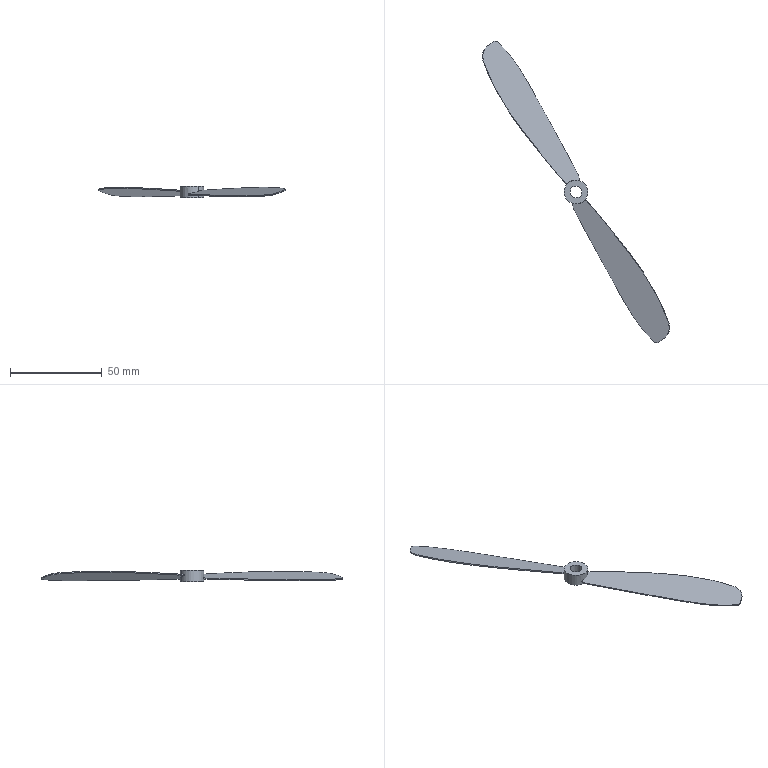Component | SolidWorks | FanBlade-3 | 1 solid | 22 faces | box 102.14 x 164.79 x 6.5 mm | volume 2171 mm3 | cylinder 8 | plane 8 | spline 6 | commonest cylinder face diameters 6.5 x2 13 x2 16 x2 4 x2
STEP:
#1=COLOUR_RGB('',0.7922,0.8196,0.9333);
#2=FILL_AREA_STYLE_COLOUR('',#1);
#3=FILL_AREA_STYLE('',(#2));
#4=SURFACE_STYLE_FILL_AREA(#3);
#5=SURFACE_SIDE_STYLE('',(#4));
#6=SURFACE_STYLE_USAGE(.BOTH.,#5);
#7=PRESENTATION_STYLE_ASSIGNMENT((#6));
#8=CARTESIAN_POINT('',(7.222,3.864,42.691));
#9=VERTEX_POINT('',#8);
#10=CARTESIAN_POINT('',(7.355,3.645,42.691));
#11=VERTEX_POINT('',#10);
#12=CARTESIAN_POINT('',(7.289,3.755,42.691));
#13=DIRECTION('',(-0.,-0.,1.));
#14=DIRECTION('',(0.521,-0.8535,0.));
#15=AXIS2_PLACEMENT_3D('',#12,#13,#14);
#16=CIRCLE('',#15,0.128);
#17=EDGE_CURVE('',#9,#11,#16,.T.);
#18=ORIENTED_EDGE('',*,*,#17,.F.);
#19=CARTESIAN_POINT('',(7.222,3.864,42.947));
#20=VERTEX_POINT('',#19);
#21=CARTESIAN_POINT('',(7.222,3.864,42.348));
#22=DIRECTION('',(-0.,-0.,1.));
#23=VECTOR('',#22,39.37);
#24=LINE('',#21,#23);
#25=EDGE_CURVE('',#9,#20,#24,.T.);
#26=ORIENTED_EDGE('',*,*,#25,.T.);
#27=CARTESIAN_POINT('',(7.355,3.645,42.947));
#28=VERTEX_POINT('',#27);
#29=CARTESIAN_POINT('',(7.289,3.755,42.947));
#30=DIRECTION('',(-0.,-0.,1.));
#31=DIRECTION('',(0.521,-0.8535,0.));
#32=AXIS2_PLACEMENT_3D('',#29,#30,#31);
#33=CIRCLE('',#32,0.128);
#34=EDGE_CURVE('',#20,#28,#33,.T.);
#35=ORIENTED_EDGE('',*,*,#34,.T.);
#36=CARTESIAN_POINT('',(7.355,3.645,42.348));
#37=DIRECTION('',(-0.,-0.,1.));
#38=VECTOR('',#37,39.37);
#39=LINE('',#36,#38);
#40=EDGE_CURVE('',#11,#28,#39,.T.);
#41=ORIENTED_EDGE('',*,*,#40,.F.);
#42=EDGE_LOOP('',(#18,#26,#35,#41));
#43=FACE_OUTER_BOUND('',#42,.T.);
#44=CARTESIAN_POINT('',(7.289,3.755,42.348));
#45=DIRECTION('',(-0.,-0.,1.));
#46=DIRECTION('',(0.521,-0.8535,0.));
#47=AXIS2_PLACEMENT_3D('',#44,#45,#46);
#48=CYLINDRICAL_SURFACE('',#47,0.128);
#49=ADVANCED_FACE('',(#43),#48,.F.);
#50=CARTESIAN_POINT('',(7.422,3.536,42.947));
#51=VERTEX_POINT('',#50);
#52=CARTESIAN_POINT('',(7.155,3.973,42.947));
#53=VERTEX_POINT('',#52);
#54=CARTESIAN_POINT('',(7.289,3.755,42.947));
#55=DIRECTION('',(-0.,-0.,1.));
#56=DIRECTION('',(0.521,-0.8535,0.));
#57=AXIS2_PLACEMENT_3D('',#54,#55,#56);
#58=CIRCLE('',#57,0.2559);
#59=EDGE_CURVE('',#51,#53,#58,.T.);
#60=ORIENTED_EDGE('',*,*,#59,.F.);
#61=CARTESIAN_POINT('',(7.422,3.536,42.831));
#62=VERTEX_POINT('',#61);
#63=CARTESIAN_POINT('',(7.422,3.536,42.947));
#64=DIRECTION('',(0.,0.,-1.));
#65=VECTOR('',#64,39.37);
#66=LINE('',#63,#65);
#67=EDGE_CURVE('',#51,#62,#66,.T.);
#68=ORIENTED_EDGE('',*,*,#67,.T.);
#69=CARTESIAN_POINT('',(7.48,3.585,42.851));
#70=VERTEX_POINT('',#69);
#71=CARTESIAN_POINT('',(7.422,3.536,42.831));
#72=CARTESIAN_POINT('',(7.444,3.55,42.838));
#73=CARTESIAN_POINT('',(7.463,3.566,42.845));
#74=CARTESIAN_POINT('',(7.48,3.585,42.851));
#75=(BOUNDED_CURVE()B_SPLINE_CURVE(3,(#71,#72,#73,#74),.UNSPECIFIED.,.F.,.F.)B_SPLINE_CURVE_WITH_KNOTS((4,4),(1.571,1.87),.UNSPECIFIED.)CURVE()GEOMETRIC_REPRESENTATION_ITEM()RATIONAL_B_SPLINE_CURVE((1.,0.9926,0.9926,1.))REPRESENTATION_ITEM(''));
#76=EDGE_CURVE('',#62,#70,#75,.T.);
#77=ORIENTED_EDGE('',*,*,#76,.T.);
#78=CARTESIAN_POINT('',(7.484,3.59,42.828));
#79=VERTEX_POINT('',#78);
#80=CARTESIAN_POINT('',(7.484,3.59,42.828));
#81=CARTESIAN_POINT('',(7.483,3.588,42.836));
#82=CARTESIAN_POINT('',(7.482,3.587,42.844));
#83=CARTESIAN_POINT('',(7.48,3.585,42.851));
#84=B_SPLINE_CURVE_WITH_KNOTS('',3,(#80,#81,#82,#83),.UNSPECIFIED.,.F.,.F.,(4,4),(0.,0.0006019),.UNSPECIFIED.);
#85=EDGE_CURVE('',#79,#70,#84,.T.);
#86=ORIENTED_EDGE('',*,*,#85,.F.);
#87=CARTESIAN_POINT('',(7.422,3.536,42.807));
#88=VERTEX_POINT('',#87);
#89=CARTESIAN_POINT('',(7.422,3.536,42.807));
#90=CARTESIAN_POINT('',(7.445,3.551,42.814));
#91=CARTESIAN_POINT('',(7.466,3.568,42.821));
#92=CARTESIAN_POINT('',(7.484,3.59,42.828));
#93=(BOUNDED_CURVE()B_SPLINE_CURVE(3,(#89,#90,#91,#92),.UNSPECIFIED.,.F.,.T.)B_SPLINE_CURVE_WITH_KNOTS((4,4),(1.571,1.892),.UNSPECIFIED.)CURVE()GEOMETRIC_REPRESENTATION_ITEM()RATIONAL_B_SPLINE_CURVE((1.,0.9914,0.9914,1.))REPRESENTATION_ITEM(''));
#94=EDGE_CURVE('',#88,#79,#93,.T.);
#95=ORIENTED_EDGE('',*,*,#94,.F.);
#96=CARTESIAN_POINT('',(7.422,3.536,42.691));
#97=VERTEX_POINT('',#96);
#98=CARTESIAN_POINT('',(7.422,3.536,42.947));
#99=DIRECTION('',(0.,0.,-1.));
#100=VECTOR('',#99,39.37);
#101=LINE('',#98,#100);
#102=EDGE_CURVE('',#88,#97,#101,.T.);
#103=ORIENTED_EDGE('',*,*,#102,.T.);
#104=CARTESIAN_POINT('',(7.155,3.973,42.691));
#105=VERTEX_POINT('',#104);
#106=CARTESIAN_POINT('',(7.289,3.755,42.691));
#107=DIRECTION('',(-0.,-0.,1.));
#108=DIRECTION('',(0.521,-0.8535,0.));
#109=AXIS2_PLACEMENT_3D('',#106,#107,#108);
#110=CIRCLE('',#109,0.2559);
#111=EDGE_CURVE('',#97,#105,#110,.T.);
#112=ORIENTED_EDGE('',*,*,#111,.T.);
#113=CARTESIAN_POINT('',(7.155,3.973,42.807));
#114=VERTEX_POINT('',#113);
#115=CARTESIAN_POINT('',(7.155,3.973,42.947));
#116=DIRECTION('',(0.,0.,-1.));
#117=VECTOR('',#116,39.37);
#118=LINE('',#115,#117);
#119=EDGE_CURVE('',#114,#105,#118,.T.);
#120=ORIENTED_EDGE('',*,*,#119,.F.);
#121=CARTESIAN_POINT('',(7.363,4.,42.756));
#122=VERTEX_POINT('',#121);
#123=CARTESIAN_POINT('',(7.363,4.,42.756));
#124=CARTESIAN_POINT('',(7.292,4.021,42.769));
#125=CARTESIAN_POINT('',(7.218,4.012,42.787));
#126=CARTESIAN_POINT('',(7.155,3.973,42.807));
#127=(BOUNDED_CURVE()B_SPLINE_CURVE(3,(#123,#124,#125,#126),.UNSPECIFIED.,.F.,.T.)B_SPLINE_CURVE_WITH_KNOTS((4,4),(0.7294,1.571),.UNSPECIFIED.)CURVE()GEOMETRIC_REPRESENTATION_ITEM()RATIONAL_B_SPLINE_CURVE((1.,0.9419,0.9419,1.))REPRESENTATION_ITEM(''));
#128=EDGE_CURVE('',#122,#114,#127,.T.);
#129=ORIENTED_EDGE('',*,*,#128,.F.);
#130=CARTESIAN_POINT('',(7.368,3.998,42.779));
#131=VERTEX_POINT('',#130);
#132=CARTESIAN_POINT('',(7.368,3.998,42.779));
#133=CARTESIAN_POINT('',(7.366,3.998,42.771));
#134=CARTESIAN_POINT('',(7.364,3.999,42.763));
#135=CARTESIAN_POINT('',(7.363,4.,42.756));
#136=(BOUNDED_CURVE()B_SPLINE_CURVE(3,(#132,#133,#134,#135),.UNSPECIFIED.,.F.,.T.)B_SPLINE_CURVE_WITH_KNOTS((4,4),(4.388,4.41),.UNSPECIFIED.)CURVE()GEOMETRIC_REPRESENTATION_ITEM()RATIONAL_B_SPLINE_CURVE((1.,1.,1.,1.))REPRESENTATION_ITEM(''));
#137=EDGE_CURVE('',#131,#122,#136,.T.);
#138=ORIENTED_EDGE('',*,*,#137,.F.);
#139=CARTESIAN_POINT('',(7.155,3.973,42.831));
#140=VERTEX_POINT('',#139);
#141=CARTESIAN_POINT('',(7.368,3.998,42.779));
#142=CARTESIAN_POINT('',(7.296,4.021,42.792));
#143=CARTESIAN_POINT('',(7.22,4.013,42.811));
#144=CARTESIAN_POINT('',(7.155,3.973,42.831));
#145=(BOUNDED_CURVE()B_SPLINE_CURVE(3,(#141,#142,#143,#144),.UNSPECIFIED.,.F.,.T.)B_SPLINE_CURVE_WITH_KNOTS((4,4),(0.7073,1.571),.UNSPECIFIED.)CURVE()GEOMETRIC_REPRESENTATION_ITEM()RATIONAL_B_SPLINE_CURVE((1.,0.9388,0.9388,1.))REPRESENTATION_ITEM(''));
#146=EDGE_CURVE('',#131,#140,#145,.T.);
#147=ORIENTED_EDGE('',*,*,#146,.T.);
#148=CARTESIAN_POINT('',(7.155,3.973,42.947));
#149=DIRECTION('',(0.,0.,-1.));
#150=VECTOR('',#149,39.37);
#151=LINE('',#148,#150);
#152=EDGE_CURVE('',#53,#140,#151,.T.);
#153=ORIENTED_EDGE('',*,*,#152,.F.);
#154=EDGE_LOOP('',(#60,#68,#77,#86,#95,#103,#112,#120,#129,#138,#147,#153));
#155=FACE_OUTER_BOUND('',#154,.T.);
#156=CARTESIAN_POINT('',(7.289,3.755,42.947));
#157=DIRECTION('',(0.,0.,-1.));
#158=DIRECTION('',(-0.521,0.8535,0.));
#159=AXIS2_PLACEMENT_3D('',#156,#157,#158);
#160=CYLINDRICAL_SURFACE('',#159,0.2559);
#161=ADVANCED_FACE('',(#155),#160,.T.);
#162=ORIENTED_EDGE('',*,*,#67,.F.);
#163=CARTESIAN_POINT('',(7.289,3.755,42.947));
#164=DIRECTION('',(-0.,-0.,1.));
#165=DIRECTION('',(0.521,-0.8535,0.));
#166=AXIS2_PLACEMENT_3D('',#163,#164,#165);
#167=CIRCLE('',#166,0.2559);
#168=EDGE_CURVE('',#53,#51,#167,.T.);
#169=ORIENTED_EDGE('',*,*,#168,.F.);
#170=ORIENTED_EDGE('',*,*,#152,.T.);
#171=CARTESIAN_POINT('',(7.097,3.924,42.851));
#172=VERTEX_POINT('',#171);
#173=CARTESIAN_POINT('',(7.155,3.973,42.831));
#174=CARTESIAN_POINT('',(7.133,3.96,42.838));
#175=CARTESIAN_POINT('',(7.114,3.943,42.845));
#176=CARTESIAN_POINT('',(7.097,3.924,42.851));
#177=(BOUNDED_CURVE()B_SPLINE_CURVE(3,(#173,#174,#175,#176),.UNSPECIFIED.,.F.,.F.)B_SPLINE_CURVE_WITH_KNOTS((4,4),(1.571,1.87),.UNSPECIFIED.)CURVE()GEOMETRIC_REPRESENTATION_ITEM()RATIONAL_B_SPLINE_CURVE((1.,0.9926,0.9926,1.))REPRESENTATION_ITEM(''));
#178=EDGE_CURVE('',#140,#172,#177,.T.);
#179=ORIENTED_EDGE('',*,*,#178,.T.);
#180=CARTESIAN_POINT('',(7.093,3.92,42.828));
#181=VERTEX_POINT('',#180);
#182=CARTESIAN_POINT('',(7.093,3.92,42.828));
#183=CARTESIAN_POINT('',(7.094,3.921,42.836));
#184=CARTESIAN_POINT('',(7.095,3.923,42.844));
#185=CARTESIAN_POINT('',(7.097,3.924,42.851));
#186=B_SPLINE_CURVE_WITH_KNOTS('',3,(#182,#183,#184,#185),.UNSPECIFIED.,.F.,.F.,(4,4),(0.,0.0006019),.UNSPECIFIED.);
#187=EDGE_CURVE('',#181,#172,#186,.T.);
#188=ORIENTED_EDGE('',*,*,#187,.F.);
#189=CARTESIAN_POINT('',(7.155,3.973,42.807));
#190=CARTESIAN_POINT('',(7.132,3.959,42.814));
#191=CARTESIAN_POINT('',(7.111,3.941,42.821));
#192=CARTESIAN_POINT('',(7.093,3.92,42.828));
#193=(BOUNDED_CURVE()B_SPLINE_CURVE(3,(#189,#190,#191,#192),.UNSPECIFIED.,.F.,.T.)B_SPLINE_CURVE_WITH_KNOTS((4,4),(1.571,1.892),.UNSPECIFIED.)CURVE()GEOMETRIC_REPRESENTATION_ITEM()RATIONAL_B_SPLINE_CURVE((1.,0.9914,0.9914,1.))REPRESENTATION_ITEM(''));
#194=EDGE_CURVE('',#114,#181,#193,.T.);
#195=ORIENTED_EDGE('',*,*,#194,.F.);
#196=ORIENTED_EDGE('',*,*,#119,.T.);
#197=CARTESIAN_POINT('',(7.289,3.755,42.691));
#198=DIRECTION('',(-0.,-0.,1.));
#199=DIRECTION('',(0.521,-0.8535,0.));
#200=AXIS2_PLACEMENT_3D('',#197,#198,#199);
#201=CIRCLE('',#200,0.2559);
#202=EDGE_CURVE('',#105,#97,#201,.T.);
#203=ORIENTED_EDGE('',*,*,#202,.T.);
#204=ORIENTED_EDGE('',*,*,#102,.F.);
#205=CARTESIAN_POINT('',(7.215,3.51,42.756));
#206=VERTEX_POINT('',#205);
#207=CARTESIAN_POINT('',(7.215,3.51,42.756));
#208=CARTESIAN_POINT('',(7.285,3.488,42.769));
#209=CARTESIAN_POINT('',(7.359,3.498,42.787));
#210=CARTESIAN_POINT('',(7.422,3.536,42.807));
#211=(BOUNDED_CURVE()B_SPLINE_CURVE(3,(#207,#208,#209,#210),.UNSPECIFIED.,.F.,.T.)B_SPLINE_CURVE_WITH_KNOTS((4,4),(0.7294,1.571),.UNSPECIFIED.)CURVE()GEOMETRIC_REPRESENTATION_ITEM()RATIONAL_B_SPLINE_CURVE((1.,0.9419,0.9419,1.))REPRESENTATION_ITEM(''));
#212=EDGE_CURVE('',#206,#88,#211,.T.);
#213=ORIENTED_EDGE('',*,*,#212,.F.);
#214=CARTESIAN_POINT('',(7.209,3.511,42.779));
#215=VERTEX_POINT('',#214);
#216=CARTESIAN_POINT('',(7.209,3.511,42.779));
#217=CARTESIAN_POINT('',(7.211,3.511,42.771));
#218=CARTESIAN_POINT('',(7.213,3.51,42.763));
#219=CARTESIAN_POINT('',(7.215,3.51,42.756));
#220=(BOUNDED_CURVE()B_SPLINE_CURVE(3,(#216,#217,#218,#219),.UNSPECIFIED.,.F.,.T.)B_SPLINE_CURVE_WITH_KNOTS((4,4),(4.388,4.41),.UNSPECIFIED.)CURVE()GEOMETRIC_REPRESENTATION_ITEM()RATIONAL_B_SPLINE_CURVE((1.,1.,1.,1.))REPRESENTATION_ITEM(''));
#221=EDGE_CURVE('',#215,#206,#220,.T.);
#222=ORIENTED_EDGE('',*,*,#221,.F.);
#223=CARTESIAN_POINT('',(7.209,3.511,42.779));
#224=CARTESIAN_POINT('',(7.281,3.488,42.792));
#225=CARTESIAN_POINT('',(7.357,3.497,42.811));
#226=CARTESIAN_POINT('',(7.422,3.536,42.831));
#227=(BOUNDED_CURVE()B_SPLINE_CURVE(3,(#223,#224,#225,#226),.UNSPECIFIED.,.F.,.T.)B_SPLINE_CURVE_WITH_KNOTS((4,4),(0.7073,1.571),.UNSPECIFIED.)CURVE()GEOMETRIC_REPRESENTATION_ITEM()RATIONAL_B_SPLINE_CURVE((1.,0.9388,0.9388,1.))REPRESENTATION_ITEM(''));
#228=EDGE_CURVE('',#215,#62,#227,.T.);
#229=ORIENTED_EDGE('',*,*,#228,.T.);
#230=EDGE_LOOP('',(#162,#169,#170,#179,#188,#195,#196,#203,#204,#213,#222,#229));
#231=FACE_OUTER_BOUND('',#230,.T.);
#232=CARTESIAN_POINT('',(7.289,3.755,42.947));
#233=DIRECTION('',(0.,0.,-1.));
#234=DIRECTION('',(-0.521,0.8535,0.));
#235=AXIS2_PLACEMENT_3D('',#232,#233,#234);
#236=CYLINDRICAL_SURFACE('',#235,0.2559);
#237=ADVANCED_FACE('',(#231),#236,.T.);
#238=CARTESIAN_POINT('',(7.289,3.755,42.947));
#239=DIRECTION('',(-0.,-0.,1.));
#240=DIRECTION('',(0.521,-0.8535,0.));
#241=AXIS2_PLACEMENT_3D('',#238,#239,#240);
#242=CIRCLE('',#241,0.128);
#243=EDGE_CURVE('',#28,#20,#242,.T.);
#244=ORIENTED_EDGE('',*,*,#243,.F.);
#245=ORIENTED_EDGE('',*,*,#34,.F.);
#246=EDGE_LOOP('',(#244,#245));
#247=FACE_BOUND('',#246,.T.);
#248=ORIENTED_EDGE('',*,*,#168,.T.);
#249=ORIENTED_EDGE('',*,*,#59,.T.);
#250=EDGE_LOOP('',(#248,#249));
#251=FACE_OUTER_BOUND('',#250,.T.);
#252=CARTESIAN_POINT('',(7.289,3.755,42.947));
#253=DIRECTION('',(-0.,-0.,1.));
#254=DIRECTION('',(0.521,-0.8535,0.));
#255=AXIS2_PLACEMENT_3D('',#252,#253,#254);
#256=PLANE('',#255);
#257=ADVANCED_FACE('',(#247,#251),#256,.T.);
#258=CARTESIAN_POINT('',(7.289,3.755,42.691));
#259=DIRECTION('',(-0.,-0.,1.));
#260=DIRECTION('',(0.521,-0.8535,0.));
#261=AXIS2_PLACEMENT_3D('',#258,#259,#260);
#262=CIRCLE('',#261,0.128);
#263=EDGE_CURVE('',#11,#9,#262,.T.);
#264=ORIENTED_EDGE('',*,*,#263,.T.);
#265=ORIENTED_EDGE('',*,*,#17,.T.);
#266=EDGE_LOOP('',(#264,#265));
#267=FACE_BOUND('',#266,.T.);
#268=ORIENTED_EDGE('',*,*,#202,.F.);
#269=ORIENTED_EDGE('',*,*,#111,.F.);
#270=EDGE_LOOP('',(#268,#269));
#271=FACE_OUTER_BOUND('',#270,.T.);
#272=CARTESIAN_POINT('',(7.289,3.755,42.691));
#273=DIRECTION('',(-0.,-0.,1.));
#274=DIRECTION('',(0.521,-0.8535,0.));
#275=AXIS2_PLACEMENT_3D('',#272,#273,#274);
#276=PLANE('',#275);
#277=ADVANCED_FACE('',(#267,#271),#276,.F.);
#278=CARTESIAN_POINT('',(9.29,0.9176,42.868));
#279=VERTEX_POINT('',#278);
#280=CARTESIAN_POINT('',(7.484,3.59,42.828));
#281=CARTESIAN_POINT('',(7.594,3.497,42.84));
#282=CARTESIAN_POINT('',(8.277,2.647,42.878));
#283=CARTESIAN_POINT('',(8.978,1.852,42.927));
#284=CARTESIAN_POINT('',(9.29,0.9176,42.868));
#285=B_SPLINE_CURVE_WITH_KNOTS('',3,(#280,#281,#282,#283,#284),.UNSPECIFIED.,.F.,.F.,(4,1,4),(0.05263,0.18,1.),.UNSPECIFIED.);
#286=EDGE_CURVE('',#79,#279,#285,.T.);
#287=ORIENTED_EDGE('',*,*,#286,.F.);
#288=ORIENTED_EDGE('',*,*,#85,.T.);
#289=CARTESIAN_POINT('',(9.285,0.9144,42.891));
#290=VERTEX_POINT('',#289);
#291=CARTESIAN_POINT('',(7.48,3.585,42.851));
#292=CARTESIAN_POINT('',(7.589,3.492,42.863));
#293=CARTESIAN_POINT('',(8.272,2.643,42.901));
#294=CARTESIAN_POINT('',(8.973,1.848,42.95));
#295=CARTESIAN_POINT('',(9.285,0.9144,42.891));
#296=B_SPLINE_CURVE_WITH_KNOTS('',3,(#291,#292,#293,#294,#295),.UNSPECIFIED.,.F.,.F.,(4,1,4),(0.05318,0.18,1.),.UNSPECIFIED.);
#297=EDGE_CURVE('',#70,#290,#296,.T.);
#298=ORIENTED_EDGE('',*,*,#297,.T.);
#299=CARTESIAN_POINT('',(9.29,0.9176,42.868));
#300=DIRECTION('',(-0.2209,-0.1349,0.9659));
#301=VECTOR('',#300,39.37);
#302=LINE('',#299,#301);
#303=EDGE_CURVE('',#279,#290,#302,.T.);
#304=ORIENTED_EDGE('',*,*,#303,.F.);
#305=EDGE_LOOP('',(#287,#288,#298,#304));
#306=FACE_OUTER_BOUND('',#305,.T.);
#307=CARTESIAN_POINT('',(7.469,3.602,42.827));
#308=CARTESIAN_POINT('',(7.464,3.599,42.849));
#309=CARTESIAN_POINT('',(7.586,3.507,42.84));
#310=CARTESIAN_POINT('',(7.58,3.504,42.863));
#311=CARTESIAN_POINT('',(8.272,2.651,42.878));
#312=CARTESIAN_POINT('',(8.267,2.648,42.9));
#313=CARTESIAN_POINT('',(8.978,1.852,42.927));
#314=CARTESIAN_POINT('',(8.973,1.848,42.95));
#315=CARTESIAN_POINT('',(9.29,0.9176,42.868));
#316=CARTESIAN_POINT('',(9.285,0.9144,42.891));
#317=B_SPLINE_SURFACE_WITH_KNOTS('',3,1,((#307,#308),(#309,#310),(#311,#312),(#313,#314),(#315,#316)),.UNSPECIFIED.,.F.,.F.,.F.,(4,1,4),(2,2),(0.04695,0.18,1.),(0.,1.),.UNSPECIFIED.);
#318=ADVANCED_FACE('',(#306),#317,.F.);
#319=CARTESIAN_POINT('',(8.961,0.5322,42.764));
#320=VERTEX_POINT('',#319);
#321=CARTESIAN_POINT('',(7.257,3.349,42.767));
#322=VERTEX_POINT('',#321);
#323=CARTESIAN_POINT('',(8.961,0.5322,42.764));
#324=CARTESIAN_POINT('',(8.664,0.8114,42.735));
#325=CARTESIAN_POINT('',(8.095,1.779,42.74));
#326=CARTESIAN_POINT('',(7.587,2.738,42.757));
#327=CARTESIAN_POINT('',(7.257,3.349,42.767));
#328=B_SPLINE_CURVE_WITH_KNOTS('',3,(#323,#324,#325,#326,#327),.UNSPECIFIED.,.F.,.F.,(4,1,4),(0.,0.3608,0.9726),.UNSPECIFIED.);
#329=EDGE_CURVE('',#320,#322,#328,.T.);
#330=ORIENTED_EDGE('',*,*,#329,.T.);
#331=CARTESIAN_POINT('',(7.262,3.353,42.744));
#332=VERTEX_POINT('',#331);
#333=CARTESIAN_POINT('',(7.257,3.349,42.767));
#334=CARTESIAN_POINT('',(7.258,3.35,42.76));
#335=CARTESIAN_POINT('',(7.26,3.351,42.752));
#336=CARTESIAN_POINT('',(7.262,3.353,42.744));
#337=B_SPLINE_CURVE_WITH_KNOTS('',3,(#333,#334,#335,#336),.UNSPECIFIED.,.F.,.F.,(4,4),(0.,0.0006001),.UNSPECIFIED.);
#338=EDGE_CURVE('',#322,#332,#337,.T.);
#339=ORIENTED_EDGE('',*,*,#338,.T.);
#340=CARTESIAN_POINT('',(8.967,0.5354,42.741));
#341=VERTEX_POINT('',#340);
#342=CARTESIAN_POINT('',(8.967,0.5354,42.741));
#343=CARTESIAN_POINT('',(8.669,0.8146,42.712));
#344=CARTESIAN_POINT('',(8.101,1.782,42.717));
#345=CARTESIAN_POINT('',(7.592,2.742,42.735));
#346=CARTESIAN_POINT('',(7.262,3.353,42.744));
#347=B_SPLINE_CURVE_WITH_KNOTS('',3,(#342,#343,#344,#345,#346),.UNSPECIFIED.,.F.,.F.,(4,1,4),(0.,0.3608,0.9727),.UNSPECIFIED.);
#348=EDGE_CURVE('',#341,#332,#347,.T.);
#349=ORIENTED_EDGE('',*,*,#348,.F.);
#350=CARTESIAN_POINT('',(8.967,0.5354,42.741));
#351=DIRECTION('',(-0.2209,-0.1349,0.9659));
#352=VECTOR('',#351,39.37);
#353=LINE('',#350,#352);
#354=EDGE_CURVE('',#341,#320,#353,.T.);
#355=ORIENTED_EDGE('',*,*,#354,.T.);
#356=EDGE_LOOP('',(#330,#339,#349,#355));
#357=FACE_OUTER_BOUND('',#356,.T.);
#358=CARTESIAN_POINT('',(8.967,0.5354,42.741));
#359=CARTESIAN_POINT('',(8.961,0.5322,42.764));
#360=CARTESIAN_POINT('',(8.669,0.8146,42.712));
#361=CARTESIAN_POINT('',(8.664,0.8114,42.735));
#362=CARTESIAN_POINT('',(8.097,1.788,42.717));
#363=CARTESIAN_POINT('',(8.092,1.785,42.74));
#364=CARTESIAN_POINT('',(7.586,2.753,42.735));
#365=CARTESIAN_POINT('',(7.581,2.75,42.758));
#366=CARTESIAN_POINT('',(7.252,3.37,42.745));
#367=CARTESIAN_POINT('',(7.247,3.367,42.768));
#368=B_SPLINE_SURFACE_WITH_KNOTS('',3,1,((#358,#359),(#360,#361),(#362,#363),(#364,#365),(#366,#367)),.UNSPECIFIED.,.F.,.F.,.F.,(4,1,4),(2,2),(0.,0.3608,0.9785),(0.,1.),.UNSPECIFIED.);
#369=ADVANCED_FACE('',(#357),#368,.F.);
#370=CARTESIAN_POINT('',(9.151,0.581,42.814));
#371=VERTEX_POINT('',#370);
#372=CARTESIAN_POINT('',(8.987,0.8499,42.814));
#373=DIRECTION('',(0.2209,0.1349,-0.9659));
#374=DIRECTION('',(0.8245,0.5033,0.2588));
#375=AXIS2_PLACEMENT_3D('',#372,#373,#374);
#376=CIRCLE('',#375,0.315);
#377=EDGE_CURVE('',#290,#371,#376,.T.);
#378=ORIENTED_EDGE('',*,*,#377,.T.);
#379=CARTESIAN_POINT('',(9.156,0.5842,42.791));
#380=VERTEX_POINT('',#379);
#381=CARTESIAN_POINT('',(9.156,0.5842,42.791));
#382=DIRECTION('',(-0.2209,-0.1349,0.9659));
#383=VECTOR('',#382,39.37);
#384=LINE('',#381,#383);
#385=EDGE_CURVE('',#380,#371,#384,.T.);
#386=ORIENTED_EDGE('',*,*,#385,.F.);
#387=CARTESIAN_POINT('',(8.992,0.853,42.791));
#388=DIRECTION('',(0.2209,0.1349,-0.9659));
#389=DIRECTION('',(0.8245,0.5033,0.2588));
#390=AXIS2_PLACEMENT_3D('',#387,#388,#389);
#391=CIRCLE('',#390,0.315);
#392=EDGE_CURVE('',#279,#380,#391,.T.);
#393=ORIENTED_EDGE('',*,*,#392,.F.);
#394=ORIENTED_EDGE('',*,*,#303,.T.);
#395=EDGE_LOOP('',(#378,#386,#393,#394));
#396=FACE_OUTER_BOUND('',#395,.T.);
#397=CARTESIAN_POINT('',(8.992,0.853,42.791));
#398=DIRECTION('',(-0.2209,-0.1349,0.9659));
#399=DIRECTION('',(-0.8245,-0.5033,-0.2588));
#400=AXIS2_PLACEMENT_3D('',#397,#398,#399);
#401=CYLINDRICAL_SURFACE('',#400,0.315);
#402=ADVANCED_FACE('',(#396),#401,.T.);
#403=CARTESIAN_POINT('',(9.054,0.5216,42.783));
#404=VERTEX_POINT('',#403);
#405=CARTESIAN_POINT('',(9.151,0.581,42.814));
#406=DIRECTION('',(-0.8245,-0.5033,-0.2588));
#407=VECTOR('',#406,39.37);
#408=LINE('',#405,#407);
#409=EDGE_CURVE('',#371,#404,#408,.T.);
#410=ORIENTED_EDGE('',*,*,#409,.T.);
#411=CARTESIAN_POINT('',(9.059,0.5248,42.761));
#412=VERTEX_POINT('',#411);
#413=CARTESIAN_POINT('',(9.059,0.5248,42.761));
#414=DIRECTION('',(-0.2209,-0.1349,0.9659));
#415=VECTOR('',#414,39.37);
#416=LINE('',#413,#415);
#417=EDGE_CURVE('',#412,#404,#416,.T.);
#418=ORIENTED_EDGE('',*,*,#417,.F.);
#419=CARTESIAN_POINT('',(9.156,0.5842,42.791));
#420=DIRECTION('',(-0.8245,-0.5033,-0.2588));
#421=VECTOR('',#420,39.37);
#422=LINE('',#419,#421);
#423=EDGE_CURVE('',#380,#412,#422,.T.);
#424=ORIENTED_EDGE('',*,*,#423,.F.);
#425=ORIENTED_EDGE('',*,*,#385,.T.);
#426=EDGE_LOOP('',(#410,#418,#424,#425));
#427=FACE_OUTER_BOUND('',#426,.T.);
#428=CARTESIAN_POINT('',(9.156,0.5842,42.791));
#429=DIRECTION('',(-0.521,0.8535,-0.));
#430=DIRECTION('',(-0.8535,-0.521,-0.));
#431=AXIS2_PLACEMENT_3D('',#428,#429,#430);
#432=PLANE('',#431);
#433=ADVANCED_FACE('',(#427),#432,.F.);
#434=CARTESIAN_POINT('',(9.012,0.5888,42.783));
#435=DIRECTION('',(0.2209,0.1349,-0.9659));
#436=DIRECTION('',(0.8245,0.5033,0.2588));
#437=AXIS2_PLACEMENT_3D('',#434,#435,#436);
#438=CIRCLE('',#437,0.07874);
#439=EDGE_CURVE('',#404,#320,#438,.T.);
#440=ORIENTED_EDGE('',*,*,#439,.T.);
#441=ORIENTED_EDGE('',*,*,#354,.F.);
#442=CARTESIAN_POINT('',(9.018,0.592,42.761));
#443=DIRECTION('',(0.2209,0.1349,-0.9659));
#444=DIRECTION('',(0.8245,0.5033,0.2588));
#445=AXIS2_PLACEMENT_3D('',#442,#443,#444);
#446=CIRCLE('',#445,0.07874);
#447=EDGE_CURVE('',#412,#341,#446,.T.);
#448=ORIENTED_EDGE('',*,*,#447,.F.);
#449=ORIENTED_EDGE('',*,*,#417,.T.);
#450=EDGE_LOOP('',(#440,#441,#448,#449));
#451=FACE_OUTER_BOUND('',#450,.T.);
#452=CARTESIAN_POINT('',(9.018,0.592,42.761));
#453=DIRECTION('',(-0.2209,-0.1349,0.9659));
#454=DIRECTION('',(-0.8245,-0.5033,-0.2588));
#455=AXIS2_PLACEMENT_3D('',#452,#453,#454);
#456=CYLINDRICAL_SURFACE('',#455,0.07874);
#457=ADVANCED_FACE('',(#451),#456,.T.);
#458=ORIENTED_EDGE('',*,*,#348,.T.);
#459=CARTESIAN_POINT('',(7.262,3.353,42.744));
#460=CARTESIAN_POINT('',(7.249,3.377,42.745));
#461=CARTESIAN_POINT('',(7.238,3.402,42.746));
#462=CARTESIAN_POINT('',(7.226,3.442,42.749));
#463=CARTESIAN_POINT('',(7.223,3.455,42.75));
#464=CARTESIAN_POINT('',(7.218,3.482,42.752));
#465=CARTESIAN_POINT('',(7.216,3.496,42.754));
#466=CARTESIAN_POINT('',(7.215,3.51,42.756));
#467=B_SPLINE_CURVE_WITH_KNOTS('',3,(#459,#460,#461,#462,#463,#464,#465,#466),.UNSPECIFIED.,.F.,.F.,(4,2,2,4),(0.,0.002088,0.003132,0.004176),.UNSPECIFIED.);
#468=EDGE_CURVE('',#332,#206,#467,.T.);
#469=ORIENTED_EDGE('',*,*,#468,.T.);
#470=ORIENTED_EDGE('',*,*,#212,.T.);
#471=ORIENTED_EDGE('',*,*,#94,.T.);
#472=ORIENTED_EDGE('',*,*,#286,.T.);
#473=ORIENTED_EDGE('',*,*,#392,.T.);
#474=ORIENTED_EDGE('',*,*,#423,.T.);
#475=ORIENTED_EDGE('',*,*,#447,.T.);
#476=EDGE_LOOP('',(#458,#469,#470,#471,#472,#473,#474,#475));
#477=FACE_OUTER_BOUND('',#476,.T.);
#478=CARTESIAN_POINT('',(8.024,1.945,42.722));
#479=DIRECTION('',(-0.2209,-0.1349,0.9659));
#480=DIRECTION('',(-0.8245,-0.5033,-0.2588));
#481=AXIS2_PLACEMENT_3D('',#478,#479,#480);
#482=PLANE('',#481);
#483=ADVANCED_FACE('',(#477),#482,.F.);
#484=ORIENTED_EDGE('',*,*,#228,.F.);
#485=CARTESIAN_POINT('',(7.209,3.511,42.779));
#486=CARTESIAN_POINT('',(7.211,3.483,42.776));
#487=CARTESIAN_POINT('',(7.216,3.455,42.773));
#488=CARTESIAN_POINT('',(7.232,3.401,42.769));
#489=CARTESIAN_POINT('',(7.243,3.374,42.768));
#490=CARTESIAN_POINT('',(7.257,3.349,42.767));
#491=B_SPLINE_CURVE_WITH_KNOTS('',3,(#485,#486,#487,#488,#489,#490),.UNSPECIFIED.,.F.,.F.,(4,2,4),(0.,0.002155,0.00431),.UNSPECIFIED.);
#492=EDGE_CURVE('',#215,#322,#491,.T.);
#493=ORIENTED_EDGE('',*,*,#492,.T.);
#494=ORIENTED_EDGE('',*,*,#329,.F.);
#495=ORIENTED_EDGE('',*,*,#439,.F.);
#496=ORIENTED_EDGE('',*,*,#409,.F.);
#497=ORIENTED_EDGE('',*,*,#377,.F.);
#498=ORIENTED_EDGE('',*,*,#297,.F.);
#499=ORIENTED_EDGE('',*,*,#76,.F.);
#500=EDGE_LOOP('',(#484,#493,#494,#495,#496,#497,#498,#499));
#501=FACE_OUTER_BOUND('',#500,.T.);
#502=CARTESIAN_POINT('',(8.019,1.942,42.745));
#503=DIRECTION('',(-0.2209,-0.1349,0.9659));
#504=DIRECTION('',(-0.8245,-0.5033,-0.2588));
#505=AXIS2_PLACEMENT_3D('',#502,#503,#504);
#506=PLANE('',#505);
#507=ADVANCED_FACE('',(#501),#506,.T.);
#508=CARTESIAN_POINT('',(5.287,6.592,42.868));
#509=VERTEX_POINT('',#508);
#510=CARTESIAN_POINT('',(7.093,3.92,42.828));
#511=CARTESIAN_POINT('',(6.983,4.013,42.84));
#512=CARTESIAN_POINT('',(6.3,4.863,42.878));
#513=CARTESIAN_POINT('',(5.599,5.658,42.927));
#514=CARTESIAN_POINT('',(5.287,6.592,42.868));
#515=B_SPLINE_CURVE_WITH_KNOTS('',3,(#510,#511,#512,#513,#514),.UNSPECIFIED.,.F.,.F.,(4,1,4),(0.05263,0.18,1.),.UNSPECIFIED.);
#516=EDGE_CURVE('',#181,#509,#515,.T.);
#517=ORIENTED_EDGE('',*,*,#516,.F.);
#518=ORIENTED_EDGE('',*,*,#187,.T.);
#519=CARTESIAN_POINT('',(5.292,6.595,42.891));
#520=VERTEX_POINT('',#519);
#521=CARTESIAN_POINT('',(7.097,3.924,42.851));
#522=CARTESIAN_POINT('',(6.988,4.017,42.863));
#523=CARTESIAN_POINT('',(6.305,4.866,42.901));
#524=CARTESIAN_POINT('',(5.604,5.661,42.95));
#525=CARTESIAN_POINT('',(5.292,6.595,42.891));
#526=B_SPLINE_CURVE_WITH_KNOTS('',3,(#521,#522,#523,#524,#525),.UNSPECIFIED.,.F.,.F.,(4,1,4),(0.05318,0.18,1.),.UNSPECIFIED.);
#527=EDGE_CURVE('',#172,#520,#526,.T.);
#528=ORIENTED_EDGE('',*,*,#527,.T.);
#529=CARTESIAN_POINT('',(5.287,6.592,42.868));
#530=DIRECTION('',(0.2209,0.1349,0.9659));
#531=VECTOR('',#530,39.37);
#532=LINE('',#529,#531);
#533=EDGE_CURVE('',#509,#520,#532,.T.);
#534=ORIENTED_EDGE('',*,*,#533,.F.);
#535=EDGE_LOOP('',(#517,#518,#528,#534));
#536=FACE_OUTER_BOUND('',#535,.T.);
#537=CARTESIAN_POINT('',(7.108,3.907,42.827));
#538=CARTESIAN_POINT('',(7.113,3.911,42.849));
#539=CARTESIAN_POINT('',(6.991,4.002,42.84));
#540=CARTESIAN_POINT('',(6.997,4.006,42.863));
#541=CARTESIAN_POINT('',(6.305,4.858,42.878));
#542=CARTESIAN_POINT('',(6.31,4.861,42.9));
#543=CARTESIAN_POINT('',(5.599,5.658,42.927));
#544=CARTESIAN_POINT('',(5.604,5.661,42.95));
#545=CARTESIAN_POINT('',(5.287,6.592,42.868));
#546=CARTESIAN_POINT('',(5.292,6.595,42.891));
#547=B_SPLINE_SURFACE_WITH_KNOTS('',3,1,((#537,#538),(#539,#540),(#541,#542),(#543,#544),(#545,#546)),.UNSPECIFIED.,.F.,.F.,.F.,(4,1,4),(2,2),(0.04695,0.18,1.),(0.,1.),.UNSPECIFIED.);
#548=ADVANCED_FACE('',(#536),#547,.F.);
#549=CARTESIAN_POINT('',(5.616,6.977,42.764));
#550=VERTEX_POINT('',#549);
#551=CARTESIAN_POINT('',(7.32,4.16,42.767));
#552=VERTEX_POINT('',#551);
#553=CARTESIAN_POINT('',(5.616,6.977,42.764));
#554=CARTESIAN_POINT('',(5.913,6.698,42.735));
#555=CARTESIAN_POINT('',(6.482,5.731,42.74));
#556=CARTESIAN_POINT('',(6.99,4.771,42.757));
#557=CARTESIAN_POINT('',(7.32,4.16,42.767));
#558=B_SPLINE_CURVE_WITH_KNOTS('',3,(#553,#554,#555,#556,#557),.UNSPECIFIED.,.F.,.F.,(4,1,4),(0.,0.3608,0.9726),.UNSPECIFIED.);
#559=EDGE_CURVE('',#550,#552,#558,.T.);
#560=ORIENTED_EDGE('',*,*,#559,.T.);
#561=CARTESIAN_POINT('',(7.315,4.157,42.744));
#562=VERTEX_POINT('',#561);
#563=CARTESIAN_POINT('',(7.32,4.16,42.767));
#564=CARTESIAN_POINT('',(7.319,4.159,42.76));
#565=CARTESIAN_POINT('',(7.317,4.158,42.752));
#566=CARTESIAN_POINT('',(7.315,4.157,42.744));
#567=B_SPLINE_CURVE_WITH_KNOTS('',3,(#563,#564,#565,#566),.UNSPECIFIED.,.F.,.F.,(4,4),(0.,0.0006001),.UNSPECIFIED.);
#568=EDGE_CURVE('',#552,#562,#567,.T.);
#569=ORIENTED_EDGE('',*,*,#568,.T.);
#570=CARTESIAN_POINT('',(5.61,6.974,42.741));
#571=VERTEX_POINT('',#570);
#572=CARTESIAN_POINT('',(5.61,6.974,42.741));
#573=CARTESIAN_POINT('',(5.908,6.695,42.712));
#574=CARTESIAN_POINT('',(6.476,5.727,42.717));
#575=CARTESIAN_POINT('',(6.985,4.768,42.735));
#576=CARTESIAN_POINT('',(7.315,4.157,42.744));
#577=B_SPLINE_CURVE_WITH_KNOTS('',3,(#572,#573,#574,#575,#576),.UNSPECIFIED.,.F.,.F.,(4,1,4),(0.,0.3608,0.9727),.UNSPECIFIED.);
#578=EDGE_CURVE('',#571,#562,#577,.T.);
#579=ORIENTED_EDGE('',*,*,#578,.F.);
#580=CARTESIAN_POINT('',(5.61,6.974,42.741));
#581=DIRECTION('',(0.2209,0.1349,0.9659));
#582=VECTOR('',#581,39.37);
#583=LINE('',#580,#582);
#584=EDGE_CURVE('',#571,#550,#583,.T.);
#585=ORIENTED_EDGE('',*,*,#584,.T.);
#586=EDGE_LOOP('',(#560,#569,#579,#585));
#587=FACE_OUTER_BOUND('',#586,.T.);
#588=CARTESIAN_POINT('',(5.61,6.974,42.741));
#589=CARTESIAN_POINT('',(5.616,6.977,42.764));
#590=CARTESIAN_POINT('',(5.908,6.695,42.712));
#591=CARTESIAN_POINT('',(5.913,6.698,42.735));
#592=CARTESIAN_POINT('',(6.48,5.721,42.717));
#593=CARTESIAN_POINT('',(6.485,5.725,42.74));
#594=CARTESIAN_POINT('',(6.991,4.756,42.735));
#595=CARTESIAN_POINT('',(6.996,4.759,42.758));
#596=CARTESIAN_POINT('',(7.325,4.139,42.745));
#597=CARTESIAN_POINT('',(7.33,4.142,42.768));
#598=B_SPLINE_SURFACE_WITH_KNOTS('',3,1,((#588,#589),(#590,#591),(#592,#593),(#594,#595),(#596,#597)),.UNSPECIFIED.,.F.,.F.,.F.,(4,1,4),(2,2),(0.,0.3608,0.9785),(0.,1.),.UNSPECIFIED.);
#599=ADVANCED_FACE('',(#587),#598,.F.);
#600=CARTESIAN_POINT('',(5.426,6.928,42.814));
#601=VERTEX_POINT('',#600);
#602=CARTESIAN_POINT('',(5.59,6.659,42.814));
#603=DIRECTION('',(-0.2209,-0.1349,-0.9659));
#604=DIRECTION('',(-0.8245,-0.5033,0.2588));
#605=AXIS2_PLACEMENT_3D('',#602,#603,#604);
#606=CIRCLE('',#605,0.315);
#607=EDGE_CURVE('',#520,#601,#606,.T.);
#608=ORIENTED_EDGE('',*,*,#607,.T.);
#609=CARTESIAN_POINT('',(5.421,6.925,42.791));
#610=VERTEX_POINT('',#609);
#611=CARTESIAN_POINT('',(5.421,6.925,42.791));
#612=DIRECTION('',(0.2209,0.1349,0.9659));
#613=VECTOR('',#612,39.37);
#614=LINE('',#611,#613);
#615=EDGE_CURVE('',#610,#601,#614,.T.);
#616=ORIENTED_EDGE('',*,*,#615,.F.);
#617=CARTESIAN_POINT('',(5.585,6.656,42.791));
#618=DIRECTION('',(-0.2209,-0.1349,-0.9659));
#619=DIRECTION('',(-0.8245,-0.5033,0.2588));
#620=AXIS2_PLACEMENT_3D('',#617,#618,#619);
#621=CIRCLE('',#620,0.315);
#622=EDGE_CURVE('',#509,#610,#621,.T.);
#623=ORIENTED_EDGE('',*,*,#622,.F.);
#624=ORIENTED_EDGE('',*,*,#533,.T.);
#625=EDGE_LOOP('',(#608,#616,#623,#624));
#626=FACE_OUTER_BOUND('',#625,.T.);
#627=CARTESIAN_POINT('',(5.585,6.656,42.791));
#628=DIRECTION('',(0.2209,0.1349,0.9659));
#629=DIRECTION('',(-0.8245,-0.5033,0.2588));
#630=AXIS2_PLACEMENT_3D('',#627,#628,#629);
#631=CYLINDRICAL_SURFACE('',#630,0.315);
#632=ADVANCED_FACE('',(#626),#631,.T.);
#633=CARTESIAN_POINT('',(5.524,6.988,42.783));
#634=VERTEX_POINT('',#633);
#635=CARTESIAN_POINT('',(5.426,6.928,42.814));
#636=DIRECTION('',(0.8245,0.5033,-0.2588));
#637=VECTOR('',#636,39.37);
#638=LINE('',#635,#637);
#639=EDGE_CURVE('',#601,#634,#638,.T.);
#640=ORIENTED_EDGE('',*,*,#639,.T.);
#641=CARTESIAN_POINT('',(5.518,6.984,42.761));
#642=VERTEX_POINT('',#641);
#643=CARTESIAN_POINT('',(5.518,6.984,42.761));
#644=DIRECTION('',(0.2209,0.1349,0.9659));
#645=VECTOR('',#644,39.37);
#646=LINE('',#643,#645);
#647=EDGE_CURVE('',#642,#634,#646,.T.);
#648=ORIENTED_EDGE('',*,*,#647,.F.);
#649=CARTESIAN_POINT('',(5.421,6.925,42.791));
#650=DIRECTION('',(0.8245,0.5033,-0.2588));
#651=VECTOR('',#650,39.37);
#652=LINE('',#649,#651);
#653=EDGE_CURVE('',#610,#642,#652,.T.);
#654=ORIENTED_EDGE('',*,*,#653,.F.);
#655=ORIENTED_EDGE('',*,*,#615,.T.);
#656=EDGE_LOOP('',(#640,#648,#654,#655));
#657=FACE_OUTER_BOUND('',#656,.T.);
#658=CARTESIAN_POINT('',(5.421,6.925,42.791));
#659=DIRECTION('',(0.521,-0.8535,0.));
#660=DIRECTION('',(0.8535,0.521,0.));
#661=AXIS2_PLACEMENT_3D('',#658,#659,#660);
#662=PLANE('',#661);
#663=ADVANCED_FACE('',(#657),#662,.F.);
#664=CARTESIAN_POINT('',(5.565,6.92,42.783));
#665=DIRECTION('',(-0.2209,-0.1349,-0.9659));
#666=DIRECTION('',(-0.8245,-0.5033,0.2588));
#667=AXIS2_PLACEMENT_3D('',#664,#665,#666);
#668=CIRCLE('',#667,0.07874);
#669=EDGE_CURVE('',#634,#550,#668,.T.);
#670=ORIENTED_EDGE('',*,*,#669,.T.);
#671=ORIENTED_EDGE('',*,*,#584,.F.);
#672=CARTESIAN_POINT('',(5.559,6.917,42.761));
#673=DIRECTION('',(-0.2209,-0.1349,-0.9659));
#674=DIRECTION('',(-0.8245,-0.5033,0.2588));
#675=AXIS2_PLACEMENT_3D('',#672,#673,#674);
#676=CIRCLE('',#675,0.07874);
#677=EDGE_CURVE('',#642,#571,#676,.T.);
#678=ORIENTED_EDGE('',*,*,#677,.F.);
#679=ORIENTED_EDGE('',*,*,#647,.T.);
#680=EDGE_LOOP('',(#670,#671,#678,#679));
#681=FACE_OUTER_BOUND('',#680,.T.);
#682=CARTESIAN_POINT('',(5.559,6.917,42.761));
#683=DIRECTION('',(0.2209,0.1349,0.9659));
#684=DIRECTION('',(-0.8245,-0.5033,0.2588));
#685=AXIS2_PLACEMENT_3D('',#682,#683,#684);
#686=CYLINDRICAL_SURFACE('',#685,0.07874);
#687=ADVANCED_FACE('',(#681),#686,.T.);
#688=ORIENTED_EDGE('',*,*,#578,.T.);
#689=CARTESIAN_POINT('',(7.315,4.157,42.744));
#690=CARTESIAN_POINT('',(7.329,4.132,42.745));
#691=CARTESIAN_POINT('',(7.339,4.107,42.746));
#692=CARTESIAN_POINT('',(7.351,4.067,42.749));
#693=CARTESIAN_POINT('',(7.354,4.054,42.75));
#694=CARTESIAN_POINT('',(7.359,4.027,42.752));
#695=CARTESIAN_POINT('',(7.361,4.013,42.754));
#696=CARTESIAN_POINT('',(7.363,4.,42.756));
#697=B_SPLINE_CURVE_WITH_KNOTS('',3,(#689,#690,#691,#692,#693,#694,#695,#696),.UNSPECIFIED.,.F.,.F.,(4,2,2,4),(0.,0.002088,0.003132,0.004176),.UNSPECIFIED.);
#698=EDGE_CURVE('',#562,#122,#697,.T.);
#699=ORIENTED_EDGE('',*,*,#698,.T.);
#700=ORIENTED_EDGE('',*,*,#128,.T.);
#701=ORIENTED_EDGE('',*,*,#194,.T.);
#702=ORIENTED_EDGE('',*,*,#516,.T.);
#703=ORIENTED_EDGE('',*,*,#622,.T.);
#704=ORIENTED_EDGE('',*,*,#653,.T.);
#705=ORIENTED_EDGE('',*,*,#677,.T.);
#706=EDGE_LOOP('',(#688,#699,#700,#701,#702,#703,#704,#705));
#707=FACE_OUTER_BOUND('',#706,.T.);
#708=CARTESIAN_POINT('',(6.553,5.564,42.722));
#709=DIRECTION('',(0.2209,0.1349,0.9659));
#710=DIRECTION('',(0.8245,0.5033,-0.2588));
#711=AXIS2_PLACEMENT_3D('',#708,#709,#710);
#712=PLANE('',#711);
#713=ADVANCED_FACE('',(#707),#712,.F.);
#714=ORIENTED_EDGE('',*,*,#146,.F.);
#715=CARTESIAN_POINT('',(7.368,3.998,42.779));
#716=CARTESIAN_POINT('',(7.366,4.026,42.776));
#717=CARTESIAN_POINT('',(7.361,4.054,42.773));
#718=CARTESIAN_POINT('',(7.345,4.108,42.769));
#719=CARTESIAN_POINT('',(7.334,4.135,42.768));
#720=CARTESIAN_POINT('',(7.32,4.16,42.767));
#721=B_SPLINE_CURVE_WITH_KNOTS('',3,(#715,#716,#717,#718,#719,#720),.UNSPECIFIED.,.F.,.F.,(4,2,4),(0.,0.002155,0.00431),.UNSPECIFIED.);
#722=EDGE_CURVE('',#131,#552,#721,.T.);
#723=ORIENTED_EDGE('',*,*,#722,.T.);
#724=ORIENTED_EDGE('',*,*,#559,.F.);
#725=ORIENTED_EDGE('',*,*,#669,.F.);
#726=ORIENTED_EDGE('',*,*,#639,.F.);
#727=ORIENTED_EDGE('',*,*,#607,.F.);
#728=ORIENTED_EDGE('',*,*,#527,.F.);
#729=ORIENTED_EDGE('',*,*,#178,.F.);
#730=EDGE_LOOP('',(#714,#723,#724,#725,#726,#727,#728,#729));
#731=FACE_OUTER_BOUND('',#730,.T.);
#732=CARTESIAN_POINT('',(6.558,5.568,42.745));
#733=DIRECTION('',(0.2209,0.1349,0.9659));
#734=DIRECTION('',(0.8245,0.5033,-0.2588));
#735=AXIS2_PLACEMENT_3D('',#732,#733,#734);
#736=PLANE('',#735);
#737=ADVANCED_FACE('',(#731),#736,.T.);
#738=ORIENTED_EDGE('',*,*,#468,.F.);
#739=ORIENTED_EDGE('',*,*,#338,.F.);
#740=ORIENTED_EDGE('',*,*,#492,.F.);
#741=ORIENTED_EDGE('',*,*,#221,.T.);
#742=EDGE_LOOP('',(#738,#739,#740,#741));
#743=FACE_OUTER_BOUND('',#742,.T.);
#744=CARTESIAN_POINT('',(7.208,3.512,42.782));
#745=CARTESIAN_POINT('',(7.215,3.425,42.77));
#746=CARTESIAN_POINT('',(7.257,3.349,42.767));
#747=CARTESIAN_POINT('',(7.21,3.511,42.773));
#748=CARTESIAN_POINT('',(7.217,3.426,42.761));
#749=CARTESIAN_POINT('',(7.259,3.35,42.758));
#750=CARTESIAN_POINT('',(7.213,3.51,42.764));
#751=CARTESIAN_POINT('',(7.22,3.426,42.752));
#752=CARTESIAN_POINT('',(7.261,3.352,42.749));
#753=CARTESIAN_POINT('',(7.215,3.51,42.755));
#754=CARTESIAN_POINT('',(7.222,3.427,42.744));
#755=CARTESIAN_POINT('',(7.263,3.353,42.74));
#756=(BOUNDED_SURFACE()B_SPLINE_SURFACE(3,2,((#744,#745,#746),(#747,#748,#749),(#750,#751,#752),(#753,#754,#755)),.UNSPECIFIED.,.F.,.F.,.F.)B_SPLINE_SURFACE_WITH_KNOTS((4,4),(3,3),(0.01863,0.01934),(0.,1.),.UNSPECIFIED.)GEOMETRIC_REPRESENTATION_ITEM()RATIONAL_B_SPLINE_SURFACE(((1.,0.9764,1.),(1.,0.9769,1.),(1.,0.9775,1.),(1.,0.978,1.)))REPRESENTATION_ITEM('')SURFACE());
#757=ADVANCED_FACE('',(#743),#756,.T.);
#758=ORIENTED_EDGE('',*,*,#698,.F.);
#759=ORIENTED_EDGE('',*,*,#568,.F.);
#760=ORIENTED_EDGE('',*,*,#722,.F.);
#761=ORIENTED_EDGE('',*,*,#137,.T.);
#762=EDGE_LOOP('',(#758,#759,#760,#761));
#763=FACE_OUTER_BOUND('',#762,.T.);
#764=CARTESIAN_POINT('',(7.369,3.998,42.782));
#765=CARTESIAN_POINT('',(7.362,4.084,42.77));
#766=CARTESIAN_POINT('',(7.32,4.16,42.767));
#767=CARTESIAN_POINT('',(7.367,3.998,42.773));
#768=CARTESIAN_POINT('',(7.36,4.083,42.761));
#769=CARTESIAN_POINT('',(7.318,4.159,42.758));
#770=CARTESIAN_POINT('',(7.365,3.999,42.764));
#771=CARTESIAN_POINT('',(7.357,4.083,42.752));
#772=CARTESIAN_POINT('',(7.316,4.157,42.749));
#773=CARTESIAN_POINT('',(7.362,4.,42.755));
#774=CARTESIAN_POINT('',(7.355,4.082,42.744));
#775=CARTESIAN_POINT('',(7.314,4.156,42.74));
#776=(BOUNDED_SURFACE()B_SPLINE_SURFACE(3,2,((#764,#765,#766),(#767,#768,#769),(#770,#771,#772),(#773,#774,#775)),.UNSPECIFIED.,.F.,.F.,.F.)B_SPLINE_SURFACE_WITH_KNOTS((4,4),(3,3),(0.01863,0.01934),(0.,1.),.UNSPECIFIED.)GEOMETRIC_REPRESENTATION_ITEM()RATIONAL_B_SPLINE_SURFACE(((1.,0.9764,1.),(1.,0.9769,1.),(1.,0.9775,1.),(1.,0.978,1.)))REPRESENTATION_ITEM('')SURFACE());
#777=ADVANCED_FACE('',(#763),#776,.T.);
#778=ORIENTED_EDGE('',*,*,#25,.F.);
#779=ORIENTED_EDGE('',*,*,#263,.F.);
#780=ORIENTED_EDGE('',*,*,#40,.T.);
#781=ORIENTED_EDGE('',*,*,#243,.T.);
#782=EDGE_LOOP('',(#778,#779,#780,#781));
#783=FACE_OUTER_BOUND('',#782,.T.);
#784=CARTESIAN_POINT('',(7.289,3.755,42.348));
#785=DIRECTION('',(-0.,-0.,1.));
#786=DIRECTION('',(0.521,-0.8535,0.));
#787=AXIS2_PLACEMENT_3D('',#784,#785,#786);
#788=CYLINDRICAL_SURFACE('',#787,0.128);
#789=ADVANCED_FACE('',(#783),#788,.F.);
#790=CLOSED_SHELL('',(#49,#161,#237,#257,#277,#318,#369,#402,#433,#457,#483,#507,#548,#599,#632,#663,#687,#713,#737,#757,#777,#789));
#791=MANIFOLD_SOLID_BREP('',#790);
#792=STYLED_ITEM('',(#7),#791);
#793=PRESENTATION_LAYER_ASSIGNMENT('','',(#792));
#794=CARTESIAN_POINT('',(0.,0.,0.));
#795=DIRECTION('',(0.,0.,1.));
#796=DIRECTION('',(1.,0.,0.));
#797=AXIS2_PLACEMENT_3D('',#794,#795,#796);
#798=(LENGTH_UNIT()NAMED_UNIT(*)SI_UNIT($,.METRE.));
#799=LENGTH_MEASURE_WITH_UNIT(LENGTH_MEASURE(0.0254),#798);
#800=DIMENSIONAL_EXPONENTS(1.,0.,0.,0.,0.,0.,0.);
#801=(CONVERSION_BASED_UNIT('',#799)LENGTH_UNIT()NAMED_UNIT(#800));
#802=UNCERTAINTY_MEASURE_WITH_UNIT(LENGTH_MEASURE(0.00001),#801,'','');
#803=(NAMED_UNIT(*)PLANE_ANGLE_UNIT()SI_UNIT($,.RADIAN.));
#804=(NAMED_UNIT(*)SI_UNIT($,.STERADIAN.)SOLID_ANGLE_UNIT());
#805=(GEOMETRIC_REPRESENTATION_CONTEXT(3)GLOBAL_UNCERTAINTY_ASSIGNED_CONTEXT((#802))GLOBAL_UNIT_ASSIGNED_CONTEXT((#801,#803,#804))REPRESENTATION_CONTEXT('',''));
#806=ADVANCED_BREP_SHAPE_REPRESENTATION('',(#791,#797),#805);
#807=(LENGTH_UNIT()NAMED_UNIT(*)SI_UNIT($,.METRE.));
#808=LENGTH_MEASURE_WITH_UNIT(LENGTH_MEASURE(0.0254),#807);
#809=DIMENSIONAL_EXPONENTS(1.,0.,0.,0.,0.,0.,0.);
#810=(CONVERSION_BASED_UNIT('',#808)LENGTH_UNIT()NAMED_UNIT(#809));
#811=UNCERTAINTY_MEASURE_WITH_UNIT(LENGTH_MEASURE(0.00001),#810,'','');
#812=(NAMED_UNIT(*)PLANE_ANGLE_UNIT()SI_UNIT($,.RADIAN.));
#813=(NAMED_UNIT(*)SI_UNIT($,.STERADIAN.)SOLID_ANGLE_UNIT());
#814=(GEOMETRIC_REPRESENTATION_CONTEXT(3)GLOBAL_UNCERTAINTY_ASSIGNED_CONTEXT((#811))GLOBAL_UNIT_ASSIGNED_CONTEXT((#810,#812,#813))REPRESENTATION_CONTEXT('',''));
#815=MECHANICAL_DESIGN_GEOMETRIC_PRESENTATION_REPRESENTATION('',(#792),#814);